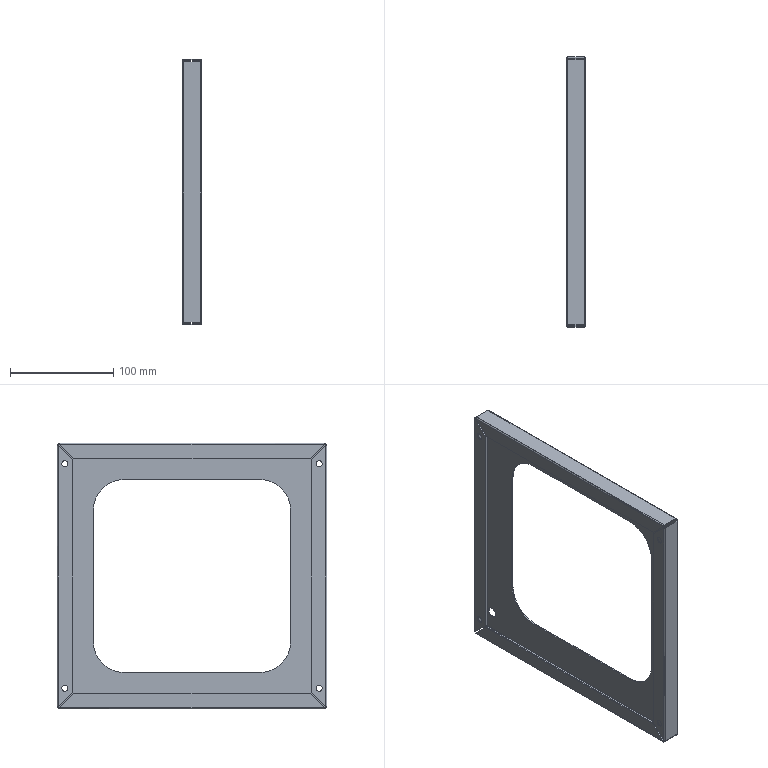Component | SolidWorks | Cover1-4XG1-1 | 1 solid | 94 faces | volume 73814 mm3 | plane 42 | cylinder 36 | spline 16 | commonest cylinder face diameters 10 x8 6 x8 2.5 x8 0.1 x8 60 x4